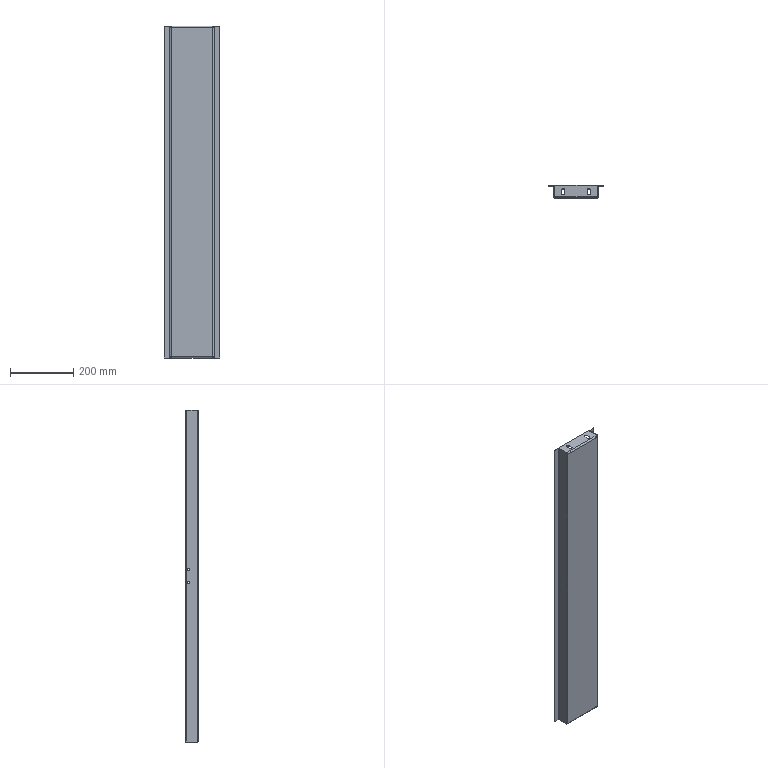Component | SolidWorks | MiddleColumn-1 | 1 solid | 78 faces | volume 536540 mm3 | plane 42 | cylinder 28 | spline 8 | commonest cylinder face diameters 7 x8 10 x8 4 x6 8 x6 | material Plain Carbon Steel